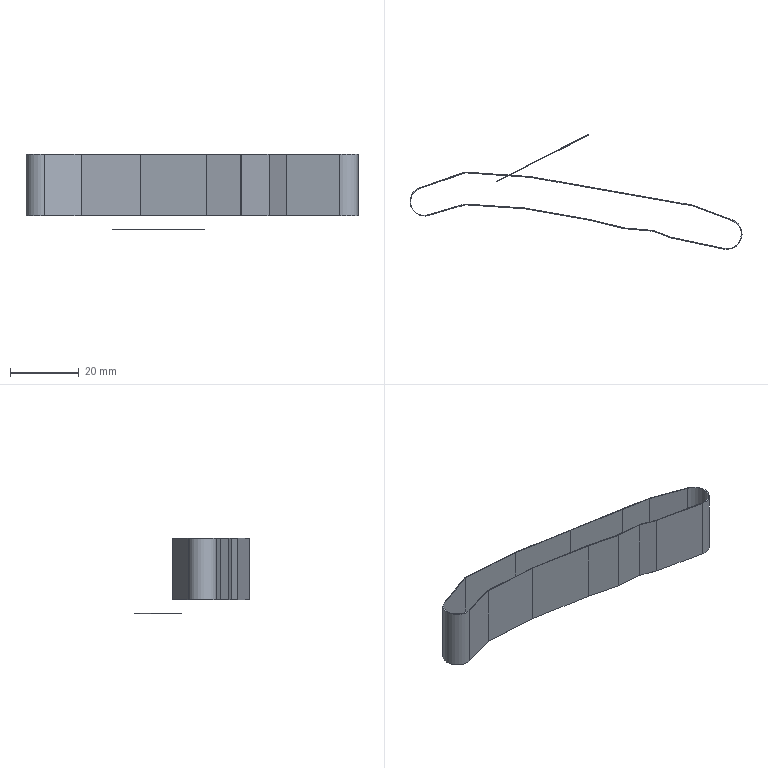Component | NX | Root-owned geometry | 2 solids | 40 faces | volume 745 mm3 | plane 30 | cylinder 9 | cone 1 | commonest cylinder face diameters 0.4 x4 8.002 x1 8.495 x1 8.402 x1 8.895 x1 0.211 x1